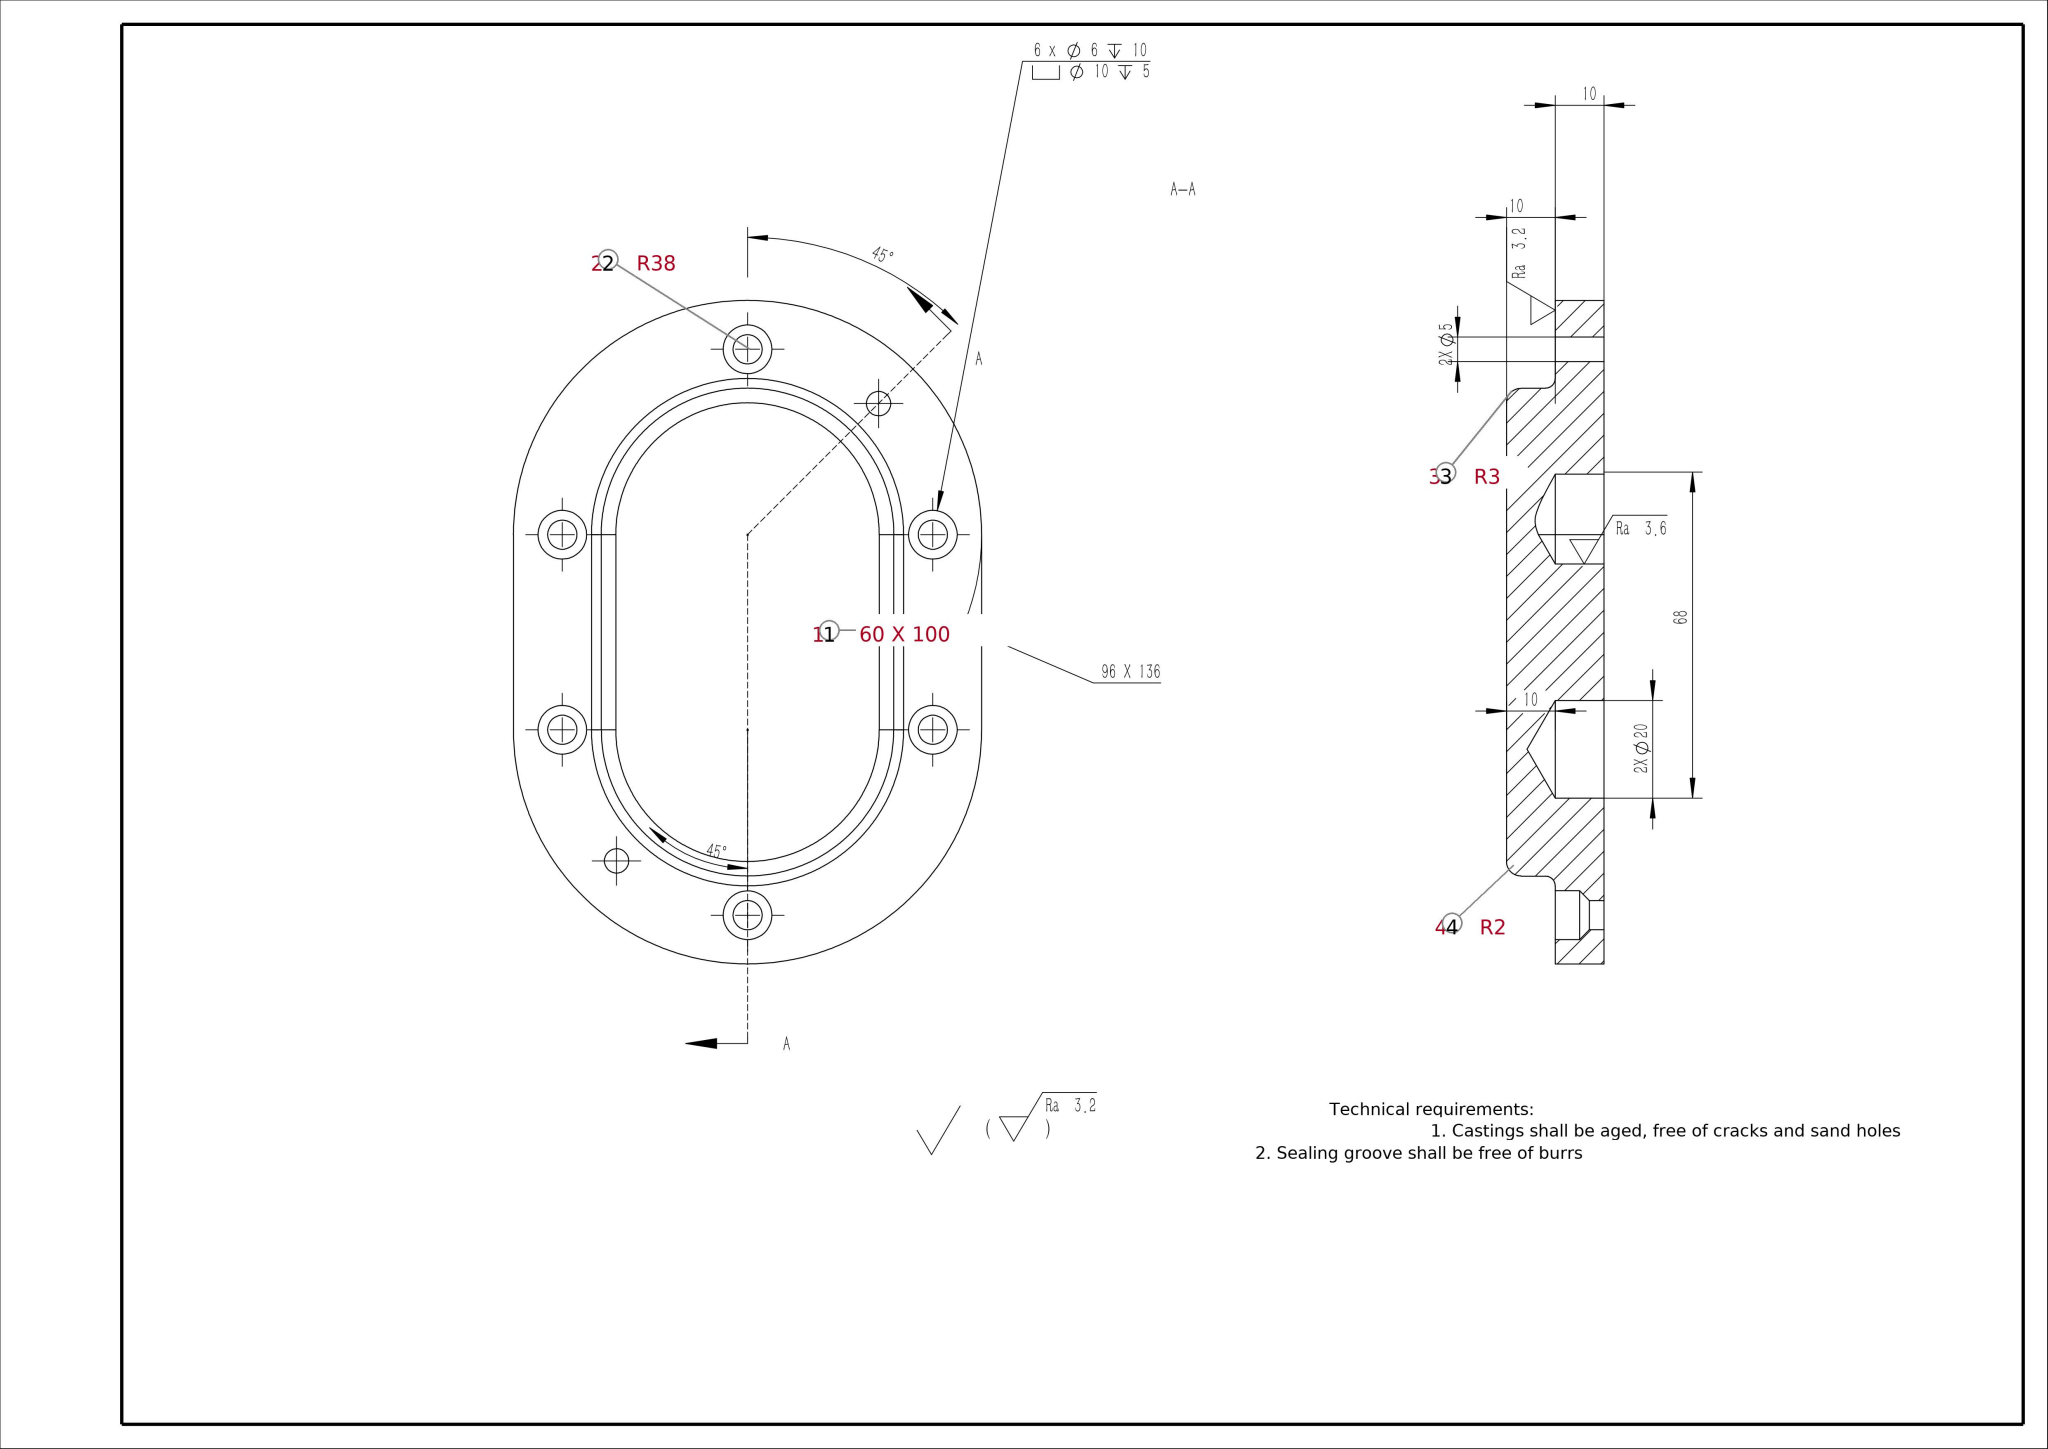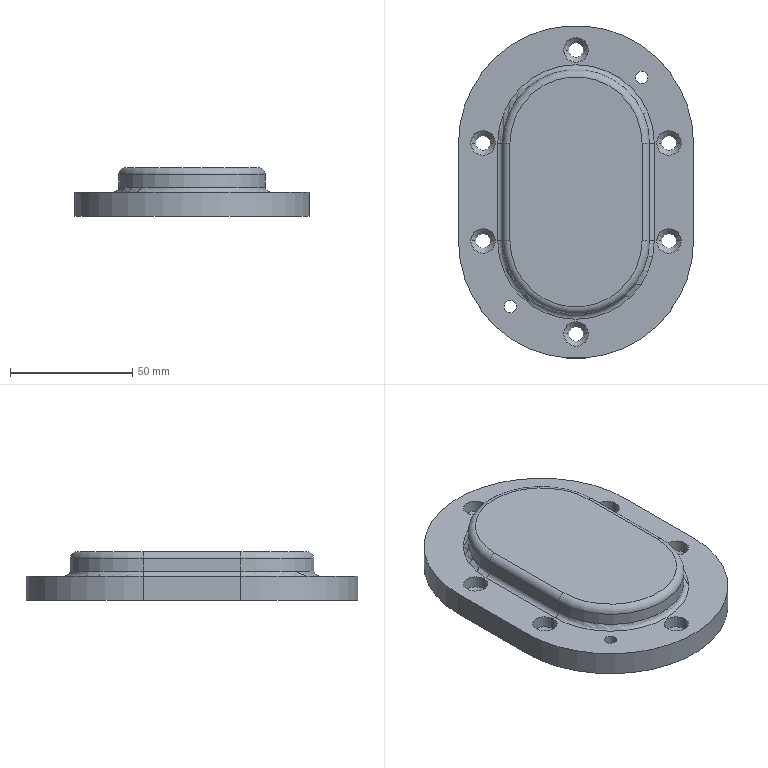Part | SolidWorks | mm | 1 solid | 67 faces | box 96 x 136 x 20 mm | volume 151413 mm3 | cylinder 40 | cone 16 | plane 7 | torus 4 | commonest cylinder face diameters 6 x14 10 x12 20 x4 5 x4 96 x2 60 x2 4 x2
build123d program:
from build123d import *

# Parameters (mm, degrees)
BOSS_EXTRUDE1_DEPTH     = 10
BOSS_EXTRUDE2_DEPTH     = 10
FILLET1_R               = 3
FILLET2_R               = 2
HOLE2_AT_2_COUNT        = 2
HOLE2_AT_2_PITCH        = 53.74
HOLE2_AT_3_COUNT        = 2
HOLE2_AT_3_PITCH        = 76
HOLE2_AT_4_COUNT        = 2
HOLE2_AT_4_PITCH        = 102.826
CUT_EXTRUDE2_DEPTH      = 10
CUT_EXTRUDE2_DEPTH_BACK = 84.833


with BuildPart() as part:
    # Sketch1 → Boss-Extrude1 (new body)
    with BuildSketch(Plane.XY):
        with BuildLine():
            Line((-48, -20), (-48, 20))
            ThreePointArc((-48, 20), (0, 68), (48, 20))
            Line((48, 20), (48, -20))
            ThreePointArc((48, -20), (0, -68), (-48, -20))
        make_face()
    extrude(amount=BOSS_EXTRUDE1_DEPTH)

    # Sketch2 → Boss-Extrude2 (add)
    with BuildSketch(Plane.XY.offset(10)):
        with BuildLine():
            Line((-30, -20), (-30, 20))
            ThreePointArc((-30, 20), (0, 50), (30, 20))
            Line((30, 20), (30, -20))
            ThreePointArc((30, -20), (0, -50), (-30, -20))
        make_face()
    extrude(amount=BOSS_EXTRUDE2_DEPTH)

    # Fillet1
    fillet1_edges = [part.edges().sort_by_distance(p)[0] for p in [
        (0, -50, 20),
        (30, 0, 20),
        (0, 50, 20),
        (-30, 0, 20),
    ]]
    fillet(fillet1_edges, radius=FILLET1_R)

    # Fillet2
    fillet2_edges = [part.edges().sort_by_distance(p)[0] for p in [
        (0, -50, 10),
        (30, 0, 10),
        (0, 50, 10),
        (-30, 0, 10),
    ]]
    fillet(fillet2_edges, radius=FILLET2_R)

    # Sketch28 → Hole2 (revolve, cut)
    with BuildSketch(Plane(origin=(38, 20, 10), x_dir=(0, -1, 0), z_dir=(1, 0, 0))):
        Polygon((0, 0), (0, 13), (3, 10), (3, 7), (5, 5), (5, 0), align=None)
    hole2 = revolve(axis=Axis((38, 20, 16.13), (0, 0, -1)), mode=Mode.SUBTRACT)

    # Hole2 at 2: Hole2 ×2
    with Locations(*[Vector(-0.7071, 0.7071, 0) * (i * HOLE2_AT_2_PITCH) for i in range(1, HOLE2_AT_2_COUNT)]):
        add(hole2, mode=Mode.SUBTRACT)

    # Hole2 at 3: Hole2 ×2
    with Locations(*[(-i * HOLE2_AT_3_PITCH, 0, 0) for i in range(1, HOLE2_AT_3_COUNT)]):
        add(hole2, mode=Mode.SUBTRACT)

    # Hole2 at 4: Hole2 ×2
    with Locations(*[Vector(0.8516, 0.5242, 0) * (i * HOLE2_AT_4_PITCH) for i in range(1, HOLE2_AT_4_COUNT)]):
        add(hole2, mode=Mode.SUBTRACT)

    # Mirror3: Hole2 across plane
    add(hole2.mirror(Plane.ZX), mode=Mode.SUBTRACT)

    # Mirror3 copy 1 sketch → Mirror3 copy 1 (revolve, cut)
    with BuildSketch(Plane(origin=(0, -58, 10), x_dir=(0, 1, 0), z_dir=(1, 0, 0))):
        Polygon((0, 0), (0, -13), (3, -10), (3, -7), (5, -5), (5, 0), align=None)
    revolve(axis=Axis((0, -58, 16.13), (0, 0, 1)), mode=Mode.SUBTRACT)

    # Mirror3 copy 2 sketch → Mirror3 copy 2 (revolve, cut)
    with BuildSketch(Plane(origin=(-38, -20, 10), x_dir=(0, 1, 0), z_dir=(1, 0, 0))):
        Polygon((0, 0), (0, -13), (3, -10), (3, -7), (5, -5), (5, 0), align=None)
    revolve(axis=Axis((-38, -20, 16.13), (0, 0, 1)), mode=Mode.SUBTRACT)

    # Mirror3 copy 3 sketch → Mirror3 copy 3 (revolve, cut)
    with BuildSketch(Plane(origin=(125.57, -73.896, 10), x_dir=(0, 1, 0), z_dir=(1, 0, 0))):
        Polygon((0, 0), (0, -13), (3, -10), (3, -7), (5, -5), (5, 0), align=None)
    revolve(axis=Axis((125.57, -73.896, 16.13), (0, 0, 1)), mode=Mode.SUBTRACT)

    # Sketch29 → Cut-Extrude2 (cut, two sides: drawn at the far end of the back side and taken through both)
    with BuildSketch(Plane.XY.offset(10).offset(-CUT_EXTRUDE2_DEPTH_BACK)):
        with BuildLine():
            ThreePointArc((-24.37, -46.87), (-24.56, -45.913), (-25.102, -45.102))
            Line((-25.102, -45.102), (-26.87, -46.87))
            ThreePointArc((-26.87, -46.87), (-25.972, -47.739), (-25.045, -48.579))
            ThreePointArc((-25.045, -48.579), (-24.545, -47.789), (-24.37, -46.87))
        make_face()
        with BuildLine():
            Line((-26.87, -46.87), (-25.102, -45.102))
            ThreePointArc((-25.102, -45.102), (-26.829, -44.37), (-28.579, -45.045))
            ThreePointArc((-28.579, -45.045), (-27.739, -45.972), (-26.87, -46.87))
        make_face()
        with BuildLine():
            ThreePointArc((-26.87, -46.87), (-27.739, -45.972), (-28.579, -45.045))
            ThreePointArc((-28.579, -45.045), (-29.37, -46.829), (-28.638, -48.638))
            Line((-28.638, -48.638), (-26.87, -46.87))
        make_face()
        with BuildLine():
            ThreePointArc((-28.638, -48.638), (-26.829, -49.37), (-25.045, -48.579))
            ThreePointArc((-25.045, -48.579), (-25.972, -47.739), (-26.87, -46.87))
            Line((-26.87, -46.87), (-28.638, -48.638))
        make_face()
        with BuildLine():
            ThreePointArc((-24.37, -46.87), (-24.56, -45.913), (-25.102, -45.102))
            Line((-25.102, -45.102), (-26.87, -46.87))
            ThreePointArc((-26.87, -46.87), (-25.972, -47.739), (-25.045, -48.579))
            ThreePointArc((-25.045, -48.579), (-24.545, -47.789), (-24.37, -46.87))
        make_face()
        with BuildLine():
            Line((-26.87, -46.87), (-25.102, -45.102))
            ThreePointArc((-25.102, -45.102), (-26.829, -44.37), (-28.579, -45.045))
            ThreePointArc((-28.579, -45.045), (-27.739, -45.972), (-26.87, -46.87))
        make_face()
        with BuildLine():
            ThreePointArc((-26.87, -46.87), (-27.739, -45.972), (-28.579, -45.045))
            ThreePointArc((-28.579, -45.045), (-29.37, -46.829), (-28.638, -48.638))
            Line((-28.638, -48.638), (-26.87, -46.87))
        make_face()
        with BuildLine():
            ThreePointArc((-28.638, -48.638), (-26.829, -49.37), (-25.045, -48.579))
            ThreePointArc((-25.045, -48.579), (-25.972, -47.739), (-26.87, -46.87))
            Line((-26.87, -46.87), (-28.638, -48.638))
        make_face()
        with BuildLine():
            ThreePointArc((-24.37, -46.87), (-24.56, -45.913), (-25.102, -45.102))
            Line((-25.102, -45.102), (-26.87, -46.87))
            ThreePointArc((-26.87, -46.87), (-25.972, -47.739), (-25.045, -48.579))
            ThreePointArc((-25.045, -48.579), (-24.545, -47.789), (-24.37, -46.87))
        make_face()
        with BuildLine():
            Line((-26.87, -46.87), (-25.102, -45.102))
            ThreePointArc((-25.102, -45.102), (-26.829, -44.37), (-28.579, -45.045))
            ThreePointArc((-28.579, -45.045), (-27.739, -45.972), (-26.87, -46.87))
        make_face()
        with BuildLine():
            ThreePointArc((-26.87, -46.87), (-27.739, -45.972), (-28.579, -45.045))
            ThreePointArc((-28.579, -45.045), (-29.37, -46.829), (-28.638, -48.638))
            Line((-28.638, -48.638), (-26.87, -46.87))
        make_face()
        with BuildLine():
            ThreePointArc((-28.638, -48.638), (-26.829, -49.37), (-25.045, -48.579))
            ThreePointArc((-25.045, -48.579), (-25.972, -47.739), (-26.87, -46.87))
            Line((-26.87, -46.87), (-28.638, -48.638))
        make_face()
        with BuildLine():
            ThreePointArc((-24.37, -46.87), (-24.56, -45.913), (-25.102, -45.102))
            Line((-25.102, -45.102), (-26.87, -46.87))
            ThreePointArc((-26.87, -46.87), (-25.972, -47.739), (-25.045, -48.579))
            ThreePointArc((-25.045, -48.579), (-24.545, -47.789), (-24.37, -46.87))
        make_face()
        with BuildLine():
            Line((-26.87, -46.87), (-25.102, -45.102))
            ThreePointArc((-25.102, -45.102), (-26.829, -44.37), (-28.579, -45.045))
            ThreePointArc((-28.579, -45.045), (-27.739, -45.972), (-26.87, -46.87))
        make_face()
        with BuildLine():
            ThreePointArc((-26.87, -46.87), (-27.739, -45.972), (-28.579, -45.045))
            ThreePointArc((-28.579, -45.045), (-29.37, -46.829), (-28.638, -48.638))
            Line((-28.638, -48.638), (-26.87, -46.87))
        make_face()
        with BuildLine():
            ThreePointArc((-28.638, -48.638), (-26.829, -49.37), (-25.045, -48.579))
            ThreePointArc((-25.045, -48.579), (-25.972, -47.739), (-26.87, -46.87))
            Line((-26.87, -46.87), (-28.638, -48.638))
        make_face()
        with BuildLine():
            ThreePointArc((28.638, 48.638), (25.102, 48.638), (25.102, 45.102))
            Line((25.102, 45.102), (28.638, 48.638))
        make_face()
        with BuildLine():
            Line((28.638, 48.638), (25.102, 45.102))
            ThreePointArc((25.102, 45.102), (27.827, 44.56), (29.37, 46.87))
            ThreePointArc((29.37, 46.87), (29.18, 47.827), (28.638, 48.638))
        make_face()
        with BuildLine():
            ThreePointArc((28.638, 48.638), (25.102, 48.638), (25.102, 45.102))
            Line((25.102, 45.102), (28.638, 48.638))
        make_face()
        with BuildLine():
            Line((28.638, 48.638), (25.102, 45.102))
            ThreePointArc((25.102, 45.102), (27.827, 44.56), (29.37, 46.87))
            ThreePointArc((29.37, 46.87), (29.18, 47.827), (28.638, 48.638))
        make_face()
    extrude(amount=CUT_EXTRUDE2_DEPTH + CUT_EXTRUDE2_DEPTH_BACK, mode=Mode.SUBTRACT)

    # Sketch30 → Cut-Revolve1 (revolve, cut)
    with BuildSketch(Plane(origin=(0, 0, 0), x_dir=(0, 0, -1), z_dir=(1, 0, 0)), mode=Mode.PRIVATE) as cut_revolve1_sk:
        Polygon((-10, 34), (-15.774, 24), (0, 24), (0, 34), align=None)
    cut_revolve1 = revolve(cut_revolve1_sk.sketch.rotate(Axis((0, 24, 77.349), (0, 0, -1)), 90), axis=Axis((0, 24, 77.349), (0, 0, -1)), mode=Mode.SUBTRACT)

    # Mirror4: Cut-Revolve1 across plane
    add(cut_revolve1.mirror(Plane.ZX), mode=Mode.SUBTRACT)


solid = part.part